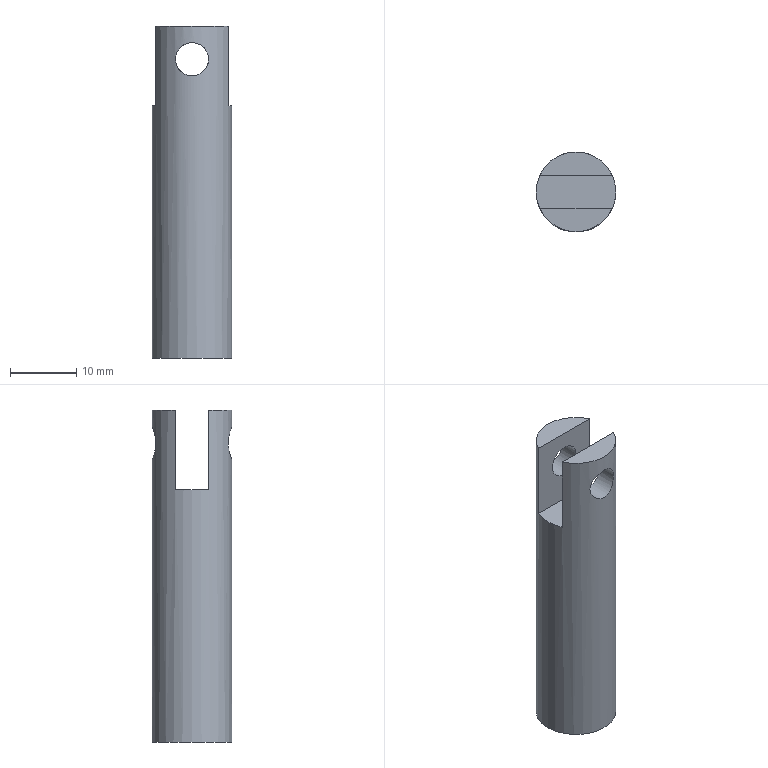Component | NX | SLIDE_ROD | 1 solid | 9 faces | volume 4824 mm3 | plane 6 | cylinder 3 | commonest cylinder face diameters 5 x2 12 x1